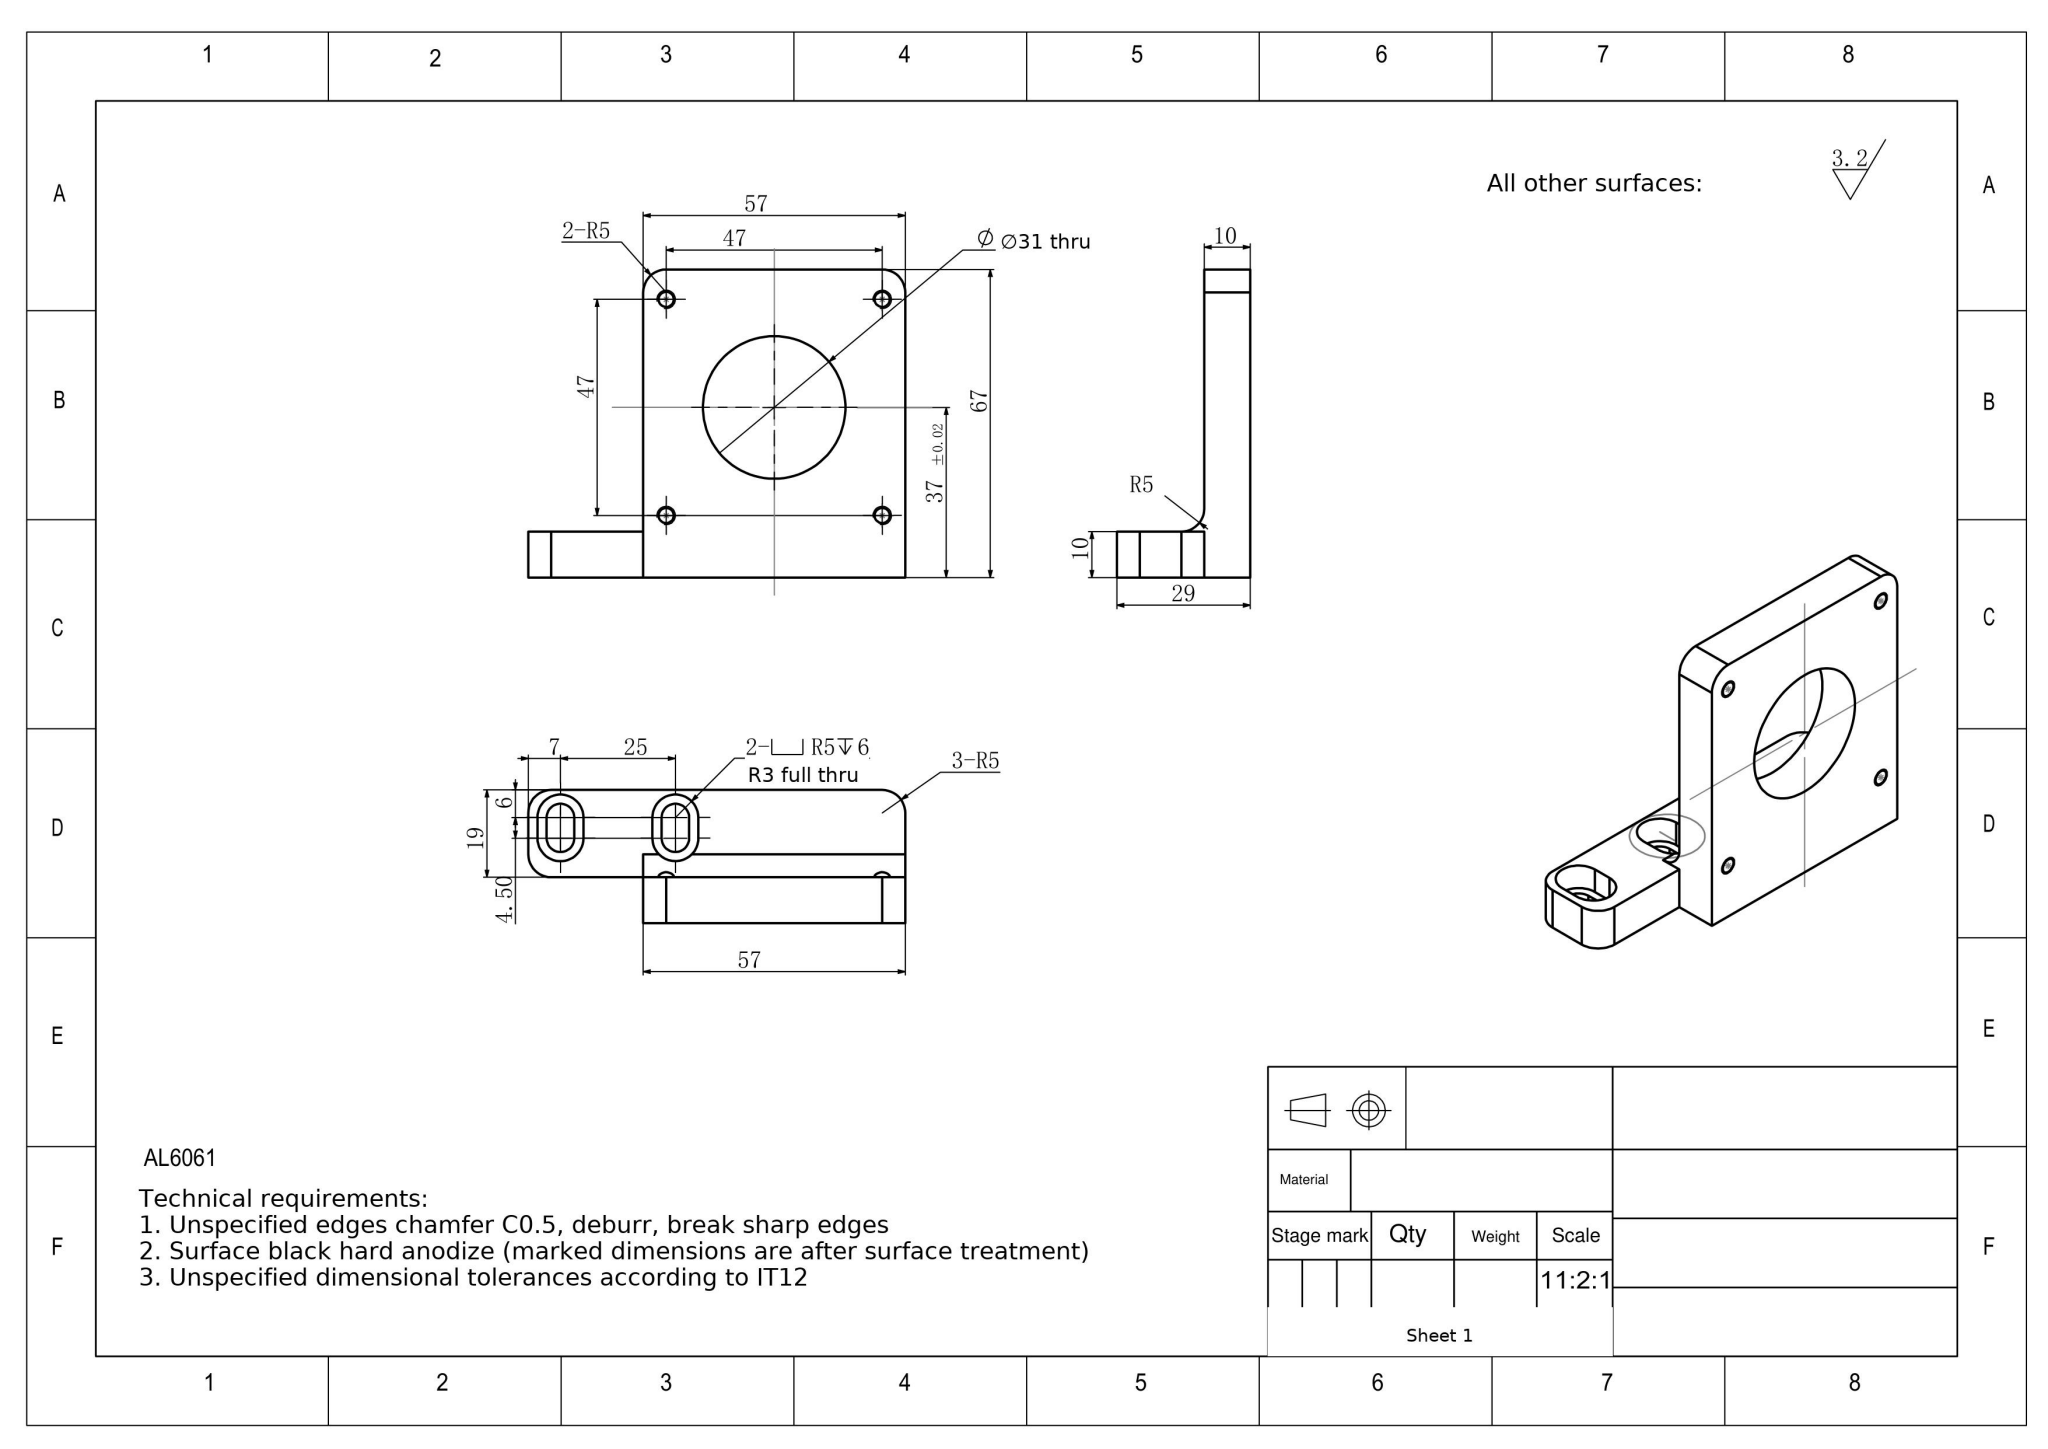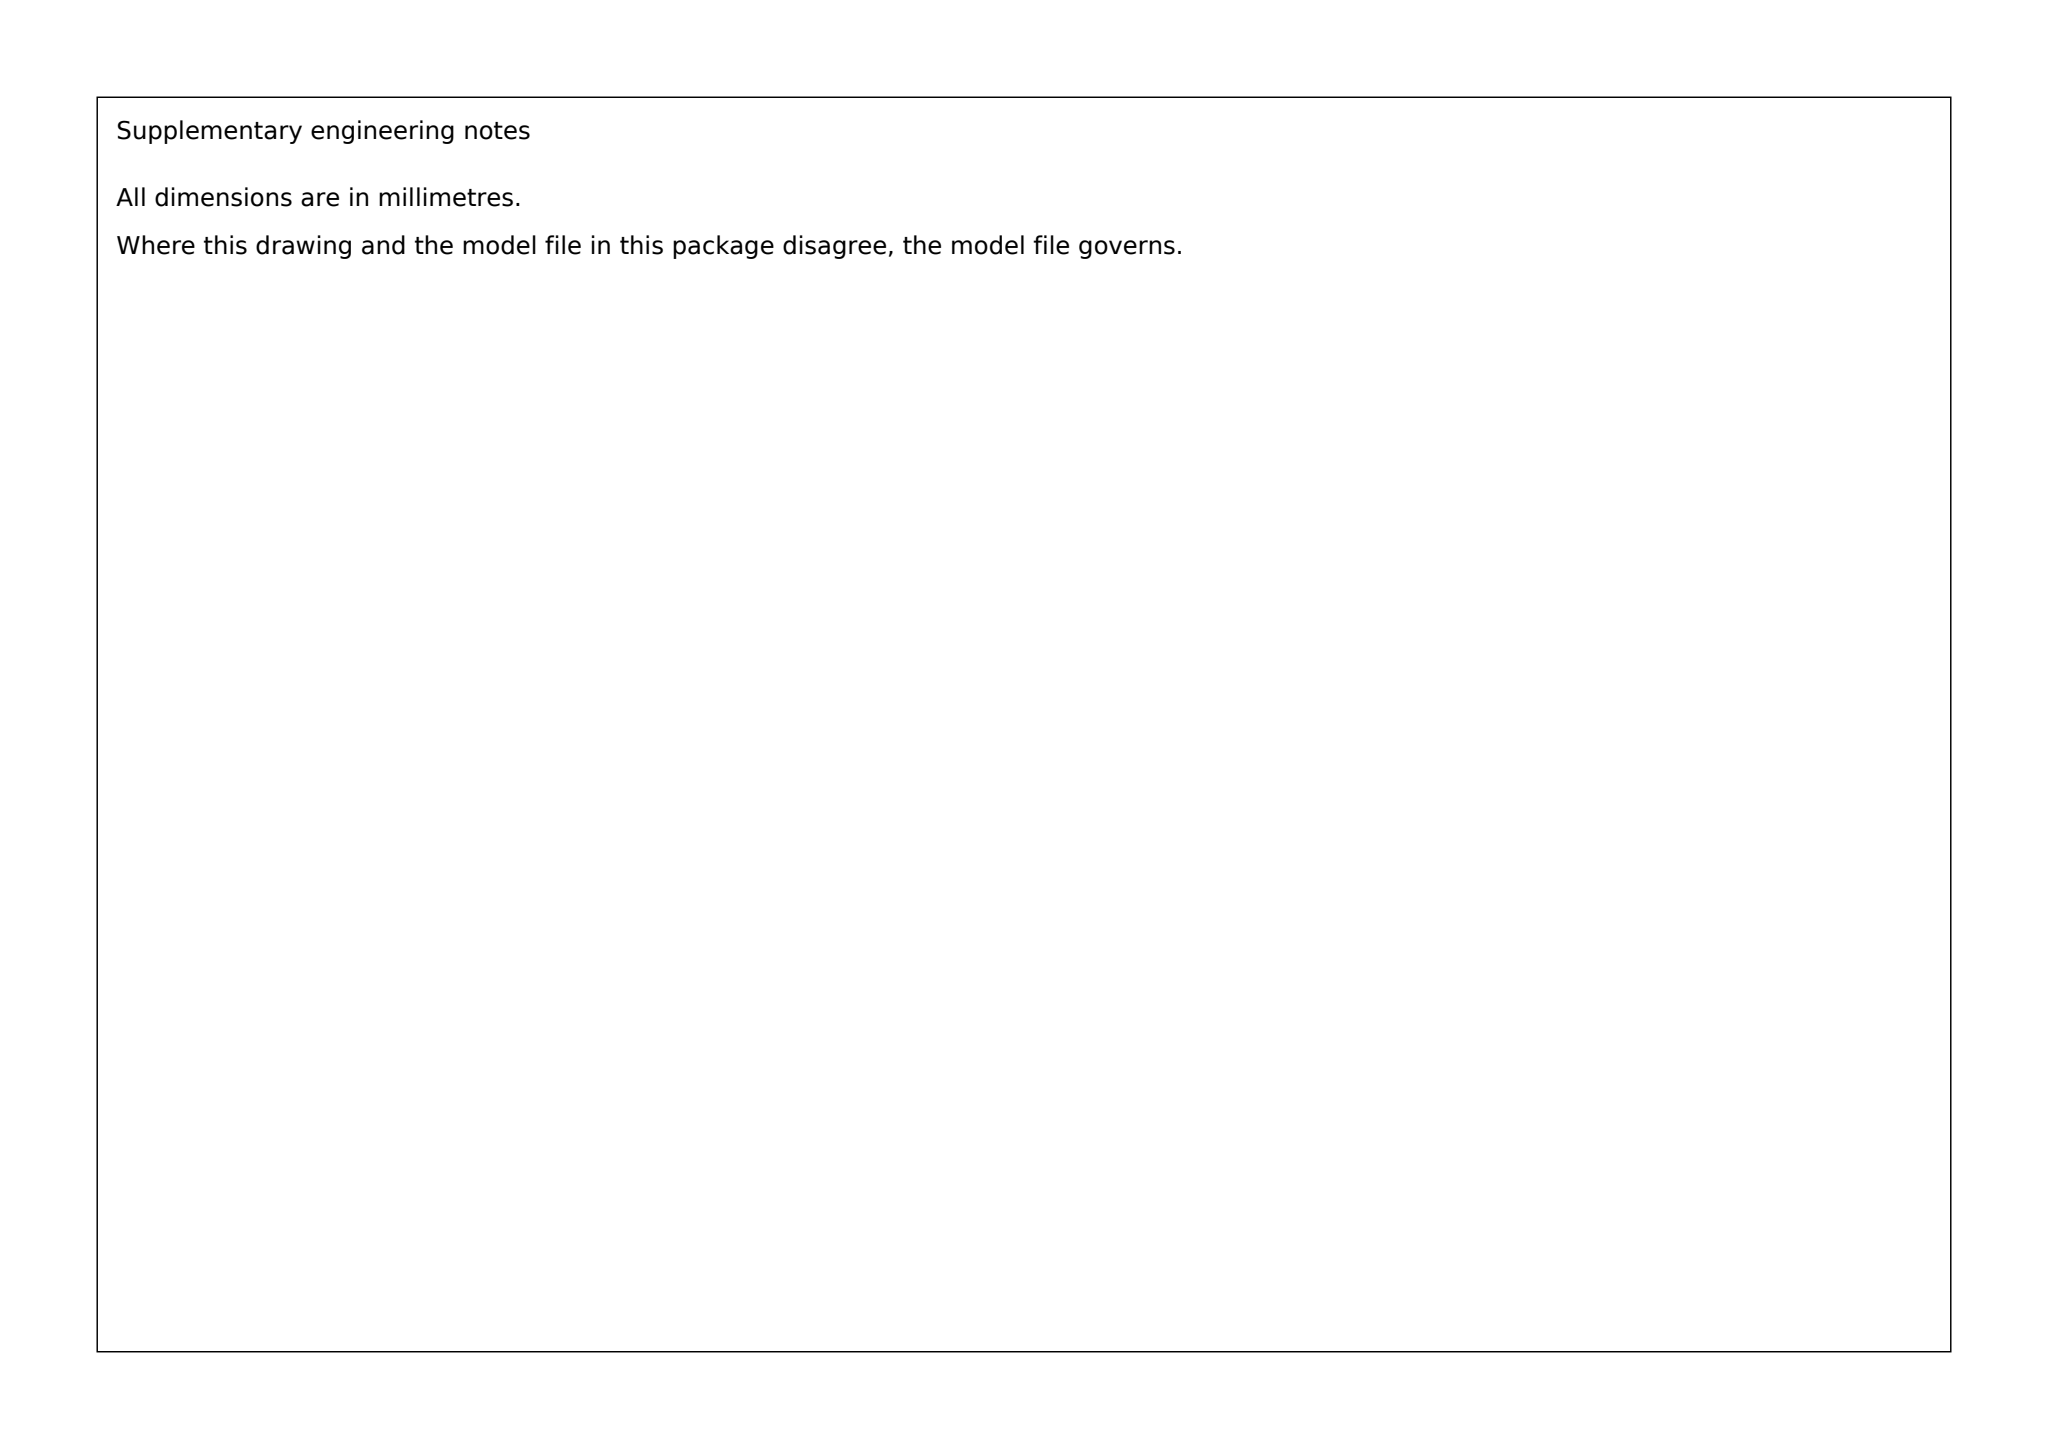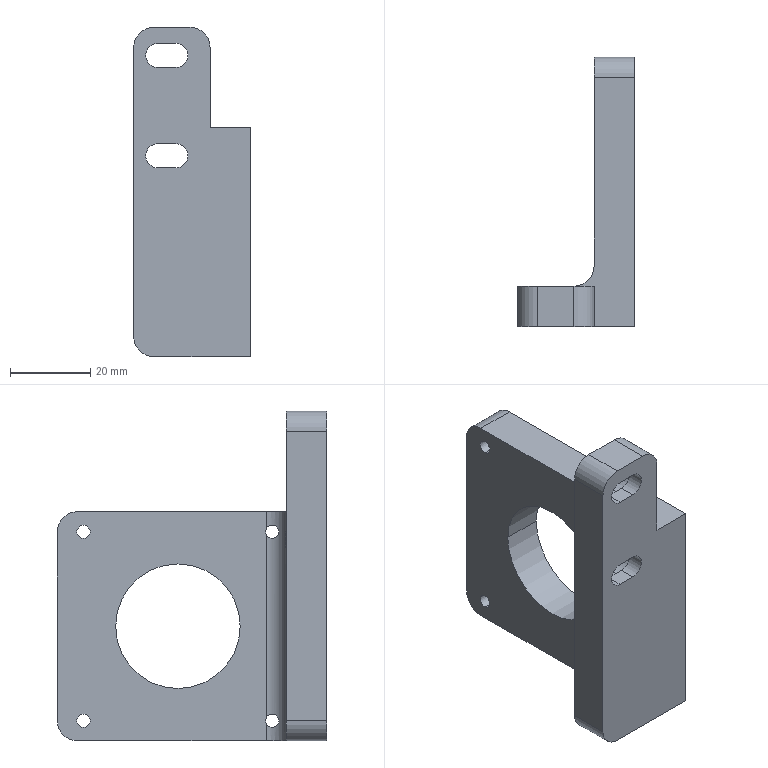Part | SolidWorks | mm | material AL6061 | 1 solid | 44 faces | box 29 x 67 x 82 mm | volume 43987 mm3 | cylinder 24 | plane 20 | commonest cylinder face diameters 10 x10 3.3 x8 6 x4 31 x2
build123d program:
from build123d import *

# Parameters (mm, degrees)
EXTRUDE1_DEPTH          = 57
FILLET1_R               = 5
SKETCH2_R               = 15.5
CUT_EXTRUDE1_DEPTH      = 85.611
M4_TAPPED_HOLE1_D       = 3.3
SKETCH6_W               = 19
SKETCH6_H               = 10
EXTRUDE2_DEPTH          = 25
FILLET2_R               = 5
CUT_EXTRUDE2_DEPTH      = 111.524
CUT_EXTRUDE3_DEPTH      = 6
CUT_EXTRUDE3_DEPTH_BACK = 6


with BuildPart() as part:
    # Sketch1 → Extrude1 (new body)
    with BuildSketch(Plane.XY):
        with BuildLine():
            Line((-18.354, 55.398), (-18.354, -11.602))
            Line((-18.354, -11.602), (-47.354, -11.602))
            Line((-47.354, -11.602), (-47.354, -1.602))
            Line((-47.354, -1.602), (-33.354, -1.602))
            ThreePointArc((-33.354, -1.602), (-29.819, -0.1375), (-28.354, 3.398))
            Line((-28.354, 3.398), (-28.354, 55.398))
            Line((-28.354, 55.398), (-18.354, 55.398))
        make_face()
    extrude(amount=EXTRUDE1_DEPTH)

    # Fillet1
    fillet1_edges = [part.edges().sort_by_distance(p)[0] for p in [
        (-23.354, 55.398, 57),
        (-47.354, -6.602, 0),
        (-23.354, 55.398, 0),
    ]]
    fillet(fillet1_edges, radius=FILLET1_R)

    # Sketch2 → Cut-Extrude1 (cut, through all)
    with BuildSketch(Plane(origin=(-18.354, 0, 0), x_dir=(0, 0, -1), z_dir=(1, 0, 0))):
        with Locations(Location((-28.5, 25.398, 0), (0, 0, 90))):
            Circle(SKETCH2_R)
    extrude(amount=-CUT_EXTRUDE1_DEPTH, mode=Mode.SUBTRACT)

    # M4 Tapped Hole1 (through all)
    with Locations(Plane(origin=(-18.354, 48.898, 52), x_dir=(0, 1, 0), z_dir=(1, 0, 0))):
        with Locations((0, 0), (0, -47), (-47, -47), (-47, 0)):
            Hole(M4_TAPPED_HOLE1_D / 2)

    # Sketch6 → Extrude2 (add)
    with BuildSketch(Plane.XY.offset(57)):
        with Locations((-37.854, -6.602)):
            Rectangle(SKETCH6_W, SKETCH6_H)
    extrude(amount=EXTRUDE2_DEPTH)

    # Fillet2
    fillet2_edges = [part.edges().sort_by_distance(p)[0] for p in [
        (-47.354, -6.602, 82),
        (-28.354, -6.602, 82),
    ]]
    fillet(fillet2_edges, radius=FILLET2_R)

    # Sketch7 → Cut-Extrude2 (cut, through all)
    with BuildSketch(Plane(origin=(0, -1.602, 0), x_dir=(1, 0, 0), z_dir=(0, 1, 0))):
        with BuildLine():
            Line((-41.354, -47), (-36.854, -47))
            ThreePointArc((-36.854, -47), (-33.854, -50), (-36.854, -53))
            Line((-36.854, -53), (-41.354, -53))
            ThreePointArc((-41.354, -53), (-44.354, -50), (-41.354, -47))
        make_face()
        with BuildLine():
            Line((-41.354, -72), (-36.854, -72))
            ThreePointArc((-36.854, -72), (-33.854, -75), (-36.854, -78))
            Line((-36.854, -78), (-41.354, -78))
            ThreePointArc((-41.354, -78), (-44.354, -75), (-41.354, -72))
        make_face()
    extrude(amount=-CUT_EXTRUDE2_DEPTH, mode=Mode.SUBTRACT)

    # Sketch8 → Cut-Extrude3 (cut, two sides: drawn at the far end of the back side and taken through both)
    with BuildSketch(Plane(origin=(0, -1.602, 0), x_dir=(1, 0, 0), z_dir=(0, 1, 0)).offset(-CUT_EXTRUDE3_DEPTH_BACK)):
        with BuildLine():
            Line((-41.354, -70), (-36.854, -70))
            ThreePointArc((-36.854, -70), (-31.854, -75), (-36.854, -80))
            Line((-36.854, -80), (-41.354, -80))
            ThreePointArc((-41.354, -80), (-46.354, -75), (-41.354, -70))
        make_face()
        with BuildLine():
            Line((-41.354, -45), (-36.854, -45))
            ThreePointArc((-36.854, -45), (-31.854, -50), (-36.854, -55))
            Line((-36.854, -55), (-41.354, -55))
            ThreePointArc((-41.354, -55), (-46.354, -50), (-41.354, -45))
        make_face()
    extrude(amount=CUT_EXTRUDE3_DEPTH + CUT_EXTRUDE3_DEPTH_BACK, mode=Mode.SUBTRACT)


solid = part.part